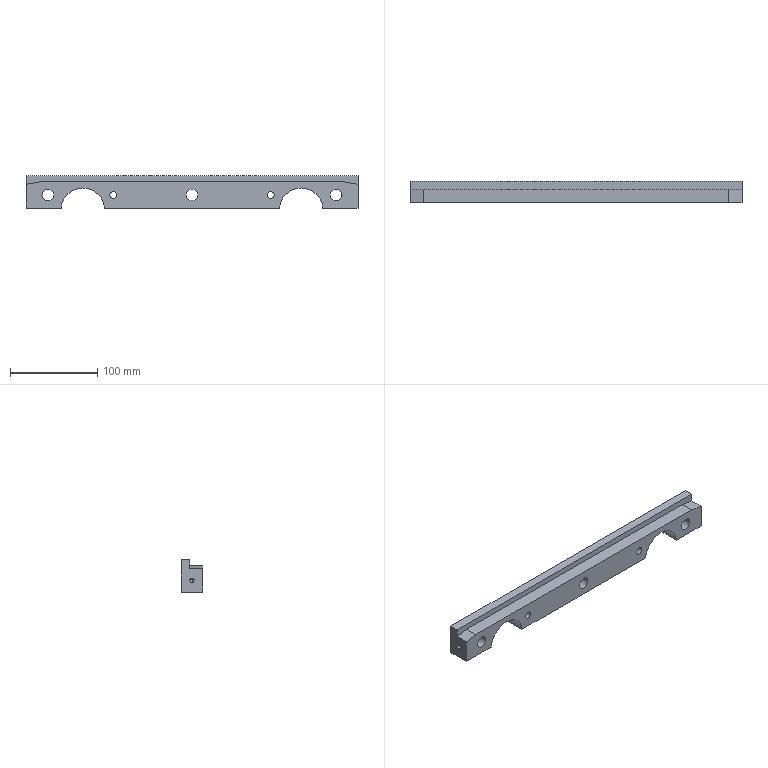Component | SolidWorks | NewDieSet-1_GuideSlot1-2 | 1 solid | 41 faces | box 380 x 25.1 x 37 mm | volume 246564 mm3 | cylinder 26 | plane 15 | commonest cylinder face diameters 5 x8 20 x6 13.5 x6 8 x4 50 x2
build123d program:
from build123d import *

# Parameters (mm, degrees)
SKETCH1_W                                            = 30
SKETCH1_H                                            = 380
BOSS_EXTRUDE1_DEPTH                                  = 25.1
SKETCH13_W                                           = 7
SKETCH13_H                                           = 10
BOSS_EXTRUDE2_DEPTH                                  = 380
HOLE_SIZE_ACCORDING_TO_HEXAGON_SOCKET_HE_D           = 13.5
HOLE_SIZE_ACCORDING_TO_HEXAGON_SOCKET_HE_CBORE_D     = 20
HOLE_SIZE_ACCORDING_TO_HEXAGON_SOCKET_HE_CBORE_DEPTH = 13
SKETCH5_R                                            = 4
CUT_EXTRUDE5_DEPTH                                   = 132
SKETCH20_R                                           = 25
CUT_EXTRUDE12_DEPTH                                  = 383.008
CHAMFER3_SIZE                                        = 15
CHAMFER3_SIZE2                                       = 2.645
M6_TAPPED_HOLE2_D                                    = 5
M6_TAPPED_HOLE2_DEPTH                                = 15
M6_TAPPED_HOLE2_TIP                                  = 1.502


with BuildPart() as part:
    # Sketch1 → Boss-Extrude1 (new body)
    with BuildSketch(Plane(origin=(0, 0, 0), x_dir=(1, 0, 0), z_dir=(0, 1, 0))):
        with Locations((-15, 190)):
            Rectangle(SKETCH1_W, SKETCH1_H)
    extrude(amount=BOSS_EXTRUDE1_DEPTH)

    # Sketch13 → Boss-Extrude2 (add)
    with BuildSketch(Plane(origin=(0, 0, -380), x_dir=(-1, 0, 0), z_dir=(0, 0, -1))):
        with Locations((-3.5, 20.1)):
            Rectangle(SKETCH13_W, SKETCH13_H)
    extrude(amount=-BOSS_EXTRUDE2_DEPTH)

    # Hole Size_According to_Hexagon Socket He (through all)
    with Locations(Plane(origin=(0, 25.1, 0), x_dir=(1, 0, 0), z_dir=(0, 1, 0))):
        with Locations((-15, 355), (-15, 25), (-15, 190)):
            CounterBoreHole(HOLE_SIZE_ACCORDING_TO_HEXAGON_SOCKET_HE_D / 2, HOLE_SIZE_ACCORDING_TO_HEXAGON_SOCKET_HE_CBORE_D / 2, HOLE_SIZE_ACCORDING_TO_HEXAGON_SOCKET_HE_CBORE_DEPTH)

    # Sketch5 → Cut-Extrude5 (cut)
    with BuildSketch(Plane.XZ):
        with Locations(Location((-15, -100, 0), (0, 0, 270))):
            Circle(SKETCH5_R)
        with Locations(Location((-15, -280, 0), (0, 0, 270))):
            Circle(SKETCH5_R)
    extrude(amount=-CUT_EXTRUDE5_DEPTH, mode=Mode.SUBTRACT)

    # Sketch20 → Cut-Extrude12 (cut, through all)
    with BuildSketch(Plane(origin=(0, 25.1, 0), x_dir=(1, 0, 0), z_dir=(0, 1, 0))):
        with Locations((-31.9, 65)):
            Circle(SKETCH20_R)
    cut_extrude12 = extrude(amount=-CUT_EXTRUDE12_DEPTH, mode=Mode.SUBTRACT)

    # Mirror2: Cut-Extrude12 across plane
    add(cut_extrude12.mirror(Plane(origin=(0, 0, -190), x_dir=(1, 0, 0), z_dir=(0, 0, -1))), mode=Mode.SUBTRACT)

    # Chamfer3
    chamfer3_edges = [part.edges().sort_by_distance(p)[0] for p in [
        (0, 7.55, 0),
        (0, 7.55, -380),
    ]]
    chamfer3_side = [part.faces().sort_by_distance(p)[0] for p in [
        (0, 7.55, -190),
    ]]
    chamfer(chamfer3_edges, length=CHAMFER3_SIZE, length2=CHAMFER3_SIZE2, reference=chamfer3_side[0])

    # Sketch21 → M6 Tapped Hole1 (revolve, cut)
    with BuildSketch(Plane(origin=(-16.322, 12.55, -380), x_dir=(0, 1, 0), z_dir=(1, 0, 0))):
        Polygon((0, 0), (0, 24.502), (2.5, 23), (2.5, 0), align=None)
    m6_tapped_hole1 = revolve(axis=Axis((-16.322, 12.55, -386.35), (0, 0, 1)), mode=Mode.SUBTRACT)

    # Mirror3: M6 Tapped Hole1 across plane
    add(m6_tapped_hole1.mirror(Plane(origin=(0, 0, -190), x_dir=(1, 0, 0), z_dir=(0, 0, -1))), mode=Mode.SUBTRACT)

    # M6 Tapped Hole2
    with Locations(Plane.ZY.offset(30)):
        with Locations((-280, 12.55), (-100, 12.55)):
            Hole(M6_TAPPED_HOLE2_D / 2, depth=M6_TAPPED_HOLE2_DEPTH)
            with Locations((0, 0, -(M6_TAPPED_HOLE2_DEPTH + M6_TAPPED_HOLE2_TIP / 2))):  # 118° drill point
                Cone(0, M6_TAPPED_HOLE2_D / 2, M6_TAPPED_HOLE2_TIP, mode=Mode.SUBTRACT)


solid = part.part

# Placed as in the assembly
solid = solid.moved(Location((-246.746, 5.927, 169.9), (0, -90, 0)))